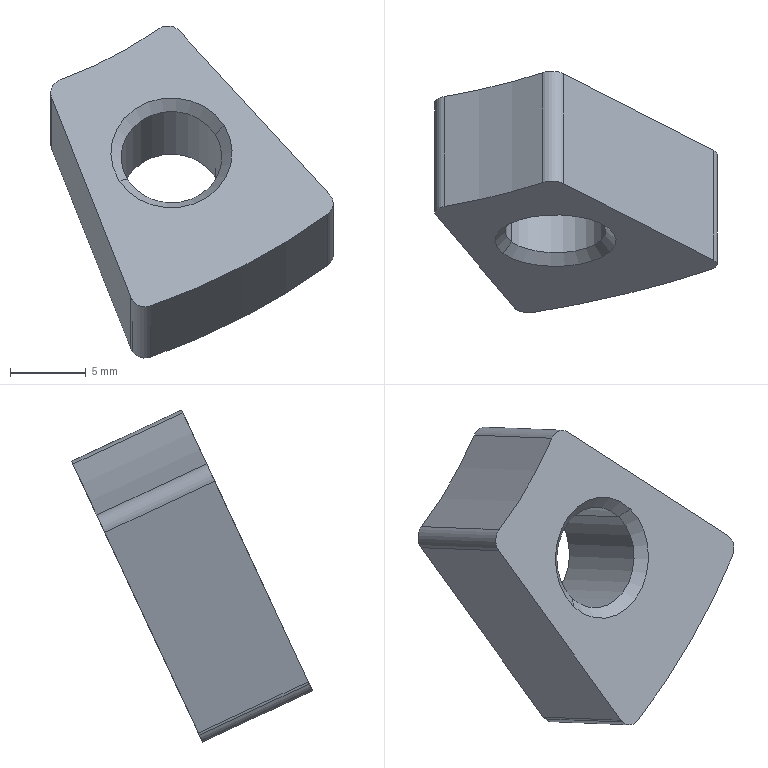Component | SolidWorks | 1369126_DSM_40_270_CC_HD_A_B_0-1_342623_DSM_40_NS-1 | 1 solid | 17 faces | box 18.64 x 15.89 x 21.91 mm | volume 1452 mm3 | cylinder 9 | cone 4 | plane 4 | commonest cylinder face diameters 2 x5 6.647 x2 89 x1 54 x1
build123d program:
from build123d import *

# Parameters (mm, degrees)
BOSS_EXTRUDE1_DEPTH = 8


with BuildPart() as part:
    # Sketch1 → Boss-Extrude1 (new body)
    with BuildSketch(Plane.XY):
        with BuildLine():
            Line((7.552, -7.828), (4.859, 7.443))
            ThreePointArc((4.859, 7.443), (4.462, 8.078), (3.736, 8.26))
            ThreePointArc((3.736, 8.26), (0, 8), (-3.736, 8.26))
            ThreePointArc((-3.736, 8.26), (-4.462, 8.078), (-4.859, 7.443))
            Line((-4.859, 7.443), (-7.552, -7.828))
            ThreePointArc((-7.552, -7.828), (-7.379, -8.584), (-6.718, -8.99))
            ThreePointArc((-6.718, -8.99), (0, -9.5), (6.718, -8.99))
            ThreePointArc((6.718, -8.99), (7.379, -8.584), (7.552, -7.828))
        make_face()
    extrude(amount=BOSS_EXTRUDE1_DEPTH)

    # Sketch2 → Cut-Revolve1 (revolve, cut)
    with BuildSketch(Plane(origin=(0, 0, 0), x_dir=(0, 0, -1), z_dir=(1, 0, 0)), mode=Mode.PRIVATE) as cut_revolve1_sk:
        Polygon((-8, 0), (-8, 4), (-7.324, 3.324), (-0.6765, 3.324), (0, 4), (0, 0), align=None)
    revolve(cut_revolve1_sk.sketch.rotate(Axis((0, 0, 0), (0, 0, 1)), 270), axis=Axis((0, 0, 0), (0, 0, 1)), mode=Mode.SUBTRACT)


solid = part.part

# Placed as in the assembly
solid = solid.moved(Location((-214.207, 2084.435, 247.117), (65, 0, 29.752)))
STEP:
#1=CARTESIAN_POINT('',(-8.547,82.013,9.681));
#2=VERTEX_POINT('',#1);
#3=CARTESIAN_POINT('',(-8.32,82.068,9.799));
#4=VERTEX_POINT('',#3);
#5=CARTESIAN_POINT('',(-8.433,82.04,9.74));
#6=DIRECTION('',(0.,-0.9063,0.4226));
#7=DIRECTION('',(0.8682,0.2097,0.4497));
#8=AXIS2_PLACEMENT_3D('',#5,#6,#7);
#9=CIRCLE('',#8,0.1308);
#10=EDGE_CURVE('',#2,#4,#9,.T.);
#11=ORIENTED_EDGE('',*,*,#10,.T.);
#12=CARTESIAN_POINT('',(-8.297,82.097,9.8));
#13=VERTEX_POINT('',#12);
#14=CARTESIAN_POINT('',(-8.297,82.097,9.8));
#15=DIRECTION('',(0.6139,0.7891,0.01917));
#16=VECTOR('',#15,39.37);
#17=LINE('',#14,#16);
#18=EDGE_CURVE('',#4,#13,#17,.T.);
#19=ORIENTED_EDGE('',*,*,#18,.T.);
#20=CARTESIAN_POINT('',(-8.57,82.031,9.658));
#21=VERTEX_POINT('',#20);
#22=CARTESIAN_POINT('',(-8.433,82.064,9.729));
#23=DIRECTION('',(0.,-0.9063,0.4226));
#24=DIRECTION('',(0.8682,0.2097,0.4497));
#25=AXIS2_PLACEMENT_3D('',#22,#23,#24);
#26=CIRCLE('',#25,0.1575);
#27=EDGE_CURVE('',#21,#13,#26,.T.);
#28=ORIENTED_EDGE('',*,*,#27,.F.);
#29=CARTESIAN_POINT('',(-8.57,82.031,9.658));
#30=DIRECTION('',(-0.6139,0.4926,-0.6168));
#31=VECTOR('',#30,39.37);
#32=LINE('',#29,#31);
#33=EDGE_CURVE('',#2,#21,#32,.T.);
#34=ORIENTED_EDGE('',*,*,#33,.F.);
#35=EDGE_LOOP('',(#11,#19,#28,#34));
#36=FACE_OUTER_BOUND('',#35,.T.);
#37=CARTESIAN_POINT('',(-8.433,82.064,9.729));
#38=DIRECTION('',(-0.,0.9063,-0.4226));
#39=DIRECTION('',(-0.8682,-0.2097,-0.4497));
#40=AXIS2_PLACEMENT_3D('',#37,#38,#39);
#41=CONICAL_SURFACE('',#40,0.1575,0.7854);
#42=ADVANCED_FACE('',(#36),#41,.F.);
#43=ORIENTED_EDGE('',*,*,#10,.F.);
#44=CARTESIAN_POINT('',(-8.547,81.776,9.792));
#45=VERTEX_POINT('',#44);
#46=CARTESIAN_POINT('',(-8.547,82.037,9.67));
#47=DIRECTION('',(0.,-0.9063,0.4226));
#48=VECTOR('',#47,39.37);
#49=LINE('',#46,#48);
#50=EDGE_CURVE('',#2,#45,#49,.T.);
#51=ORIENTED_EDGE('',*,*,#50,.T.);
#52=CARTESIAN_POINT('',(-8.32,81.83,9.91));
#53=VERTEX_POINT('',#52);
#54=CARTESIAN_POINT('',(-8.433,81.803,9.851));
#55=DIRECTION('',(0.,-0.9063,0.4226));
#56=DIRECTION('',(0.8682,0.2097,0.4497));
#57=AXIS2_PLACEMENT_3D('',#54,#55,#56);
#58=CIRCLE('',#57,0.1308);
#59=EDGE_CURVE('',#45,#53,#58,.T.);
#60=ORIENTED_EDGE('',*,*,#59,.T.);
#61=CARTESIAN_POINT('',(-8.32,82.092,9.788));
#62=DIRECTION('',(0.,-0.9063,0.4226));
#63=VECTOR('',#62,39.37);
#64=LINE('',#61,#63);
#65=EDGE_CURVE('',#4,#53,#64,.T.);
#66=ORIENTED_EDGE('',*,*,#65,.F.);
#67=EDGE_LOOP('',(#43,#51,#60,#66));
#68=FACE_OUTER_BOUND('',#67,.T.);
#69=CARTESIAN_POINT('',(-8.433,82.064,9.729));
#70=DIRECTION('',(0.,-0.9063,0.4226));
#71=DIRECTION('',(0.8682,0.2097,0.4497));
#72=AXIS2_PLACEMENT_3D('',#69,#70,#71);
#73=CYLINDRICAL_SURFACE('',#72,0.1308);
#74=ADVANCED_FACE('',(#68),#73,.F.);
#75=ORIENTED_EDGE('',*,*,#59,.F.);
#76=CARTESIAN_POINT('',(-8.57,81.746,9.791));
#77=VERTEX_POINT('',#76);
#78=CARTESIAN_POINT('',(-8.547,81.776,9.792));
#79=DIRECTION('',(-0.6139,-0.7891,-0.01917));
#80=VECTOR('',#79,39.37);
#81=LINE('',#78,#80);
#82=EDGE_CURVE('',#45,#77,#81,.T.);
#83=ORIENTED_EDGE('',*,*,#82,.T.);
#84=CARTESIAN_POINT('',(-8.297,81.812,9.933));
#85=VERTEX_POINT('',#84);
#86=CARTESIAN_POINT('',(-8.433,81.779,9.862));
#87=DIRECTION('',(0.,-0.9063,0.4226));
#88=DIRECTION('',(0.8682,0.2097,0.4497));
#89=AXIS2_PLACEMENT_3D('',#86,#87,#88);
#90=CIRCLE('',#89,0.1575);
#91=EDGE_CURVE('',#77,#85,#90,.T.);
#92=ORIENTED_EDGE('',*,*,#91,.T.);
#93=CARTESIAN_POINT('',(-8.32,81.83,9.91));
#94=DIRECTION('',(0.6139,-0.4926,0.6168));
#95=VECTOR('',#94,39.37);
#96=LINE('',#93,#95);
#97=EDGE_CURVE('',#53,#85,#96,.T.);
#98=ORIENTED_EDGE('',*,*,#97,.F.);
#99=EDGE_LOOP('',(#75,#83,#92,#98));
#100=FACE_OUTER_BOUND('',#99,.T.);
#101=CARTESIAN_POINT('',(-8.433,81.803,9.851));
#102=DIRECTION('',(0.,-0.9063,0.4226));
#103=DIRECTION('',(0.8682,0.2097,0.4497));
#104=AXIS2_PLACEMENT_3D('',#101,#102,#103);
#105=CONICAL_SURFACE('',#104,0.1308,0.7854);
#106=ADVANCED_FACE('',(#100),#105,.F.);
#107=CARTESIAN_POINT('',(-8.536,81.601,9.48));
#108=VERTEX_POINT('',#107);
#109=CARTESIAN_POINT('',(-8.487,81.594,9.465));
#110=VERTEX_POINT('',#109);
#111=CARTESIAN_POINT('',(-8.501,81.609,9.498));
#112=DIRECTION('',(0.,-0.9063,0.4226));
#113=DIRECTION('',(0.8682,0.2097,0.4497));
#114=AXIS2_PLACEMENT_3D('',#111,#112,#113);
#115=CIRCLE('',#114,0.03937);
#116=EDGE_CURVE('',#108,#110,#115,.T.);
#117=ORIENTED_EDGE('',*,*,#116,.F.);
#118=CARTESIAN_POINT('',(-8.536,81.886,9.347));
#119=VERTEX_POINT('',#118);
#120=CARTESIAN_POINT('',(-8.536,81.601,9.48));
#121=DIRECTION('',(-0.,0.9063,-0.4226));
#122=VECTOR('',#121,39.37);
#123=LINE('',#120,#122);
#124=EDGE_CURVE('',#108,#119,#123,.T.);
#125=ORIENTED_EDGE('',*,*,#124,.T.);
#126=CARTESIAN_POINT('',(-8.487,81.879,9.332));
#127=VERTEX_POINT('',#126);
#128=CARTESIAN_POINT('',(-8.501,81.895,9.365));
#129=DIRECTION('',(0.,-0.9063,0.4226));
#130=DIRECTION('',(0.8682,0.2097,0.4497));
#131=AXIS2_PLACEMENT_3D('',#128,#129,#130);
#132=CIRCLE('',#131,0.03937);
#133=EDGE_CURVE('',#119,#127,#132,.T.);
#134=ORIENTED_EDGE('',*,*,#133,.T.);
#135=CARTESIAN_POINT('',(-8.487,81.594,9.465));
#136=DIRECTION('',(-0.,0.9063,-0.4226));
#137=VECTOR('',#136,39.37);
#138=LINE('',#135,#137);
#139=EDGE_CURVE('',#110,#127,#138,.T.);
#140=ORIENTED_EDGE('',*,*,#139,.F.);
#141=EDGE_LOOP('',(#117,#125,#134,#140));
#142=FACE_OUTER_BOUND('',#141,.T.);
#143=CARTESIAN_POINT('',(-8.501,81.609,9.498));
#144=DIRECTION('',(-0.,0.9063,-0.4226));
#145=DIRECTION('',(-0.8682,-0.2097,-0.4497));
#146=AXIS2_PLACEMENT_3D('',#143,#144,#145);
#147=CYLINDRICAL_SURFACE('',#146,0.03937);
#148=ADVANCED_FACE('',(#142),#147,.T.);
#149=ORIENTED_EDGE('',*,*,#124,.F.);
#150=CARTESIAN_POINT('',(-8.539,81.603,9.486));
#151=VERTEX_POINT('',#150);
#152=CARTESIAN_POINT('',(-8.501,81.609,9.498));
#153=DIRECTION('',(0.,-0.9063,0.4226));
#154=DIRECTION('',(0.8682,0.2097,0.4497));
#155=AXIS2_PLACEMENT_3D('',#152,#153,#154);
#156=CIRCLE('',#155,0.03937);
#157=EDGE_CURVE('',#151,#108,#156,.T.);
#158=ORIENTED_EDGE('',*,*,#157,.F.);
#159=CARTESIAN_POINT('',(-8.539,81.889,9.353));
#160=VERTEX_POINT('',#159);
#161=CARTESIAN_POINT('',(-8.539,81.603,9.486));
#162=DIRECTION('',(-0.,0.9063,-0.4226));
#163=VECTOR('',#162,39.37);
#164=LINE('',#161,#163);
#165=EDGE_CURVE('',#151,#160,#164,.T.);
#166=ORIENTED_EDGE('',*,*,#165,.T.);
#167=CARTESIAN_POINT('',(-8.501,81.895,9.365));
#168=DIRECTION('',(0.,-0.9063,0.4226));
#169=DIRECTION('',(0.8682,0.2097,0.4497));
#170=AXIS2_PLACEMENT_3D('',#167,#168,#169);
#171=CIRCLE('',#170,0.03937);
#172=EDGE_CURVE('',#160,#119,#171,.T.);
#173=ORIENTED_EDGE('',*,*,#172,.T.);
#174=EDGE_LOOP('',(#149,#158,#166,#173));
#175=FACE_OUTER_BOUND('',#174,.T.);
#176=CARTESIAN_POINT('',(-8.501,81.609,9.498));
#177=DIRECTION('',(-0.,0.9063,-0.4226));
#178=DIRECTION('',(-0.8682,-0.2097,-0.4497));
#179=AXIS2_PLACEMENT_3D('',#176,#177,#178);
#180=CYLINDRICAL_SURFACE('',#179,0.03937);
#181=ADVANCED_FACE('',(#175),#180,.T.);
#182=CARTESIAN_POINT('',(-8.028,81.99,9.569));
#183=VERTEX_POINT('',#182);
#184=CARTESIAN_POINT('',(-9.117,82.57,10.813));
#185=DIRECTION('',(0.,-0.9063,0.4226));
#186=DIRECTION('',(0.8682,0.2097,0.4497));
#187=AXIS2_PLACEMENT_3D('',#184,#185,#186);
#188=CIRCLE('',#187,1.752);
#189=EDGE_CURVE('',#127,#183,#188,.T.);
#190=ORIENTED_EDGE('',*,*,#189,.T.);
#191=CARTESIAN_POINT('',(-8.028,81.705,9.703));
#192=VERTEX_POINT('',#191);
#193=CARTESIAN_POINT('',(-8.028,81.705,9.703));
#194=DIRECTION('',(-0.,0.9063,-0.4226));
#195=VECTOR('',#194,39.37);
#196=LINE('',#193,#195);
#197=EDGE_CURVE('',#192,#183,#196,.T.);
#198=ORIENTED_EDGE('',*,*,#197,.F.);
#199=CARTESIAN_POINT('',(-9.117,82.285,10.946));
#200=DIRECTION('',(0.,-0.9063,0.4226));
#201=DIRECTION('',(0.8682,0.2097,0.4497));
#202=AXIS2_PLACEMENT_3D('',#199,#200,#201);
#203=CIRCLE('',#202,1.752);
#204=EDGE_CURVE('',#110,#192,#203,.T.);
#205=ORIENTED_EDGE('',*,*,#204,.F.);
#206=ORIENTED_EDGE('',*,*,#139,.T.);
#207=EDGE_LOOP('',(#190,#198,#205,#206));
#208=FACE_OUTER_BOUND('',#207,.T.);
#209=CARTESIAN_POINT('',(-9.117,82.285,10.946));
#210=DIRECTION('',(-0.,0.9063,-0.4226));
#211=DIRECTION('',(-0.8682,-0.2097,-0.4497));
#212=AXIS2_PLACEMENT_3D('',#209,#210,#211);
#213=CYLINDRICAL_SURFACE('',#212,1.752);
#214=ADVANCED_FACE('',(#208),#213,.T.);
#215=CARTESIAN_POINT('',(-8.022,82.014,9.62));
#216=VERTEX_POINT('',#215);
#217=CARTESIAN_POINT('',(-8.053,82.003,9.597));
#218=DIRECTION('',(0.,-0.9063,0.4226));
#219=DIRECTION('',(0.8682,0.2097,0.4497));
#220=AXIS2_PLACEMENT_3D('',#217,#218,#219);
#221=CIRCLE('',#220,0.03937);
#222=EDGE_CURVE('',#183,#216,#221,.T.);
#223=ORIENTED_EDGE('',*,*,#222,.T.);
#224=CARTESIAN_POINT('',(-8.022,81.728,9.753));
#225=VERTEX_POINT('',#224);
#226=CARTESIAN_POINT('',(-8.022,81.728,9.753));
#227=DIRECTION('',(-0.,0.9063,-0.4226));
#228=VECTOR('',#227,39.37);
#229=LINE('',#226,#228);
#230=EDGE_CURVE('',#225,#216,#229,.T.);
#231=ORIENTED_EDGE('',*,*,#230,.F.);
#232=CARTESIAN_POINT('',(-8.053,81.718,9.731));
#233=DIRECTION('',(0.,-0.9063,0.4226));
#234=DIRECTION('',(0.8682,0.2097,0.4497));
#235=AXIS2_PLACEMENT_3D('',#232,#233,#234);
#236=CIRCLE('',#235,0.03937);
#237=EDGE_CURVE('',#192,#225,#236,.T.);
#238=ORIENTED_EDGE('',*,*,#237,.F.);
#239=ORIENTED_EDGE('',*,*,#197,.T.);
#240=EDGE_LOOP('',(#223,#231,#238,#239));
#241=FACE_OUTER_BOUND('',#240,.T.);
#242=CARTESIAN_POINT('',(-8.053,81.718,9.731));
#243=DIRECTION('',(-0.,0.9063,-0.4226));
#244=DIRECTION('',(-0.8682,-0.2097,-0.4497));
#245=AXIS2_PLACEMENT_3D('',#242,#243,#244);
#246=CYLINDRICAL_SURFACE('',#245,0.03937);
#247=ADVANCED_FACE('',(#241),#246,.T.);
#248=CARTESIAN_POINT('',(-8.413,82.212,10.046));
#249=VERTEX_POINT('',#248);
#250=CARTESIAN_POINT('',(-8.022,82.014,9.62));
#251=DIRECTION('',(-0.6394,0.3249,0.6968));
#252=VECTOR('',#251,39.37);
#253=LINE('',#250,#252);
#254=EDGE_CURVE('',#216,#249,#253,.T.);
#255=ORIENTED_EDGE('',*,*,#254,.T.);
#256=CARTESIAN_POINT('',(-8.413,81.927,10.179));
#257=VERTEX_POINT('',#256);
#258=CARTESIAN_POINT('',(-8.413,81.927,10.179));
#259=DIRECTION('',(-0.,0.9063,-0.4226));
#260=VECTOR('',#259,39.37);
#261=LINE('',#258,#260);
#262=EDGE_CURVE('',#257,#249,#261,.T.);
#263=ORIENTED_EDGE('',*,*,#262,.F.);
#264=CARTESIAN_POINT('',(-8.022,81.728,9.753));
#265=DIRECTION('',(-0.6394,0.3249,0.6968));
#266=VECTOR('',#265,39.37);
#267=LINE('',#264,#266);
#268=EDGE_CURVE('',#225,#257,#267,.T.);
#269=ORIENTED_EDGE('',*,*,#268,.F.);
#270=ORIENTED_EDGE('',*,*,#230,.T.);
#271=EDGE_LOOP('',(#255,#263,#269,#270));
#272=FACE_OUTER_BOUND('',#271,.T.);
#273=CARTESIAN_POINT('',(-8.022,81.728,9.753));
#274=DIRECTION('',(-0.7688,-0.2702,-0.5795));
#275=DIRECTION('',(0.6394,-0.3249,-0.6968));
#276=AXIS2_PLACEMENT_3D('',#273,#274,#275);
#277=PLANE('',#276);
#278=ADVANCED_FACE('',(#272),#277,.F.);
#279=CARTESIAN_POINT('',(-8.467,82.215,10.051));
#280=VERTEX_POINT('',#279);
#281=CARTESIAN_POINT('',(-8.443,82.201,10.023));
#282=DIRECTION('',(0.,-0.9063,0.4226));
#283=DIRECTION('',(0.8682,0.2097,0.4497));
#284=AXIS2_PLACEMENT_3D('',#281,#282,#283);
#285=CIRCLE('',#284,0.03937);
#286=EDGE_CURVE('',#249,#280,#285,.T.);
#287=ORIENTED_EDGE('',*,*,#286,.T.);
#288=CARTESIAN_POINT('',(-8.467,81.929,10.184));
#289=VERTEX_POINT('',#288);
#290=CARTESIAN_POINT('',(-8.467,81.929,10.184));
#291=DIRECTION('',(-0.,0.9063,-0.4226));
#292=VECTOR('',#291,39.37);
#293=LINE('',#290,#292);
#294=EDGE_CURVE('',#289,#280,#293,.T.);
#295=ORIENTED_EDGE('',*,*,#294,.F.);
#296=CARTESIAN_POINT('',(-8.443,81.916,10.156));
#297=DIRECTION('',(0.,-0.9063,0.4226));
#298=DIRECTION('',(0.8682,0.2097,0.4497));
#299=AXIS2_PLACEMENT_3D('',#296,#297,#298);
#300=CIRCLE('',#299,0.03937);
#301=EDGE_CURVE('',#257,#289,#300,.T.);
#302=ORIENTED_EDGE('',*,*,#301,.F.);
#303=ORIENTED_EDGE('',*,*,#262,.T.);
#304=EDGE_LOOP('',(#287,#295,#302,#303));
#305=FACE_OUTER_BOUND('',#304,.T.);
#306=CARTESIAN_POINT('',(-8.443,81.916,10.156));
#307=DIRECTION('',(-0.,0.9063,-0.4226));
#308=DIRECTION('',(-0.8682,-0.2097,-0.4497));
#309=AXIS2_PLACEMENT_3D('',#306,#307,#308);
#310=CYLINDRICAL_SURFACE('',#309,0.03937);
#311=ADVANCED_FACE('',(#305),#310,.T.);
#312=CARTESIAN_POINT('',(-8.722,82.153,9.919));
#313=VERTEX_POINT('',#312);
#314=CARTESIAN_POINT('',(-9.117,82.57,10.813));
#315=DIRECTION('',(-0.,0.9063,-0.4226));
#316=DIRECTION('',(-0.8682,-0.2097,-0.4497));
#317=AXIS2_PLACEMENT_3D('',#314,#315,#316);
#318=CIRCLE('',#317,1.063);
#319=EDGE_CURVE('',#280,#313,#318,.T.);
#320=ORIENTED_EDGE('',*,*,#319,.T.);
#321=CARTESIAN_POINT('',(-8.722,81.867,10.052));
#322=VERTEX_POINT('',#321);
#323=CARTESIAN_POINT('',(-8.722,81.867,10.052));
#324=DIRECTION('',(-0.,0.9063,-0.4226));
#325=VECTOR('',#324,39.37);
#326=LINE('',#323,#325);
#327=EDGE_CURVE('',#322,#313,#326,.T.);
#328=ORIENTED_EDGE('',*,*,#327,.F.);
#329=CARTESIAN_POINT('',(-9.117,82.285,10.946));
#330=DIRECTION('',(-0.,0.9063,-0.4226));
#331=DIRECTION('',(-0.8682,-0.2097,-0.4497));
#332=AXIS2_PLACEMENT_3D('',#329,#330,#331);
#333=CIRCLE('',#332,1.063);
#334=EDGE_CURVE('',#289,#322,#333,.T.);
#335=ORIENTED_EDGE('',*,*,#334,.F.);
#336=ORIENTED_EDGE('',*,*,#294,.T.);
#337=EDGE_LOOP('',(#320,#328,#335,#336));
#338=FACE_OUTER_BOUND('',#337,.T.);
#339=CARTESIAN_POINT('',(-9.117,82.285,10.946));
#340=DIRECTION('',(-0.,0.9063,-0.4226));
#341=DIRECTION('',(-0.8682,-0.2097,-0.4497));
#342=AXIS2_PLACEMENT_3D('',#339,#340,#341);
#343=CYLINDRICAL_SURFACE('',#342,1.063);
#344=ADVANCED_FACE('',(#338),#343,.F.);
#345=CARTESIAN_POINT('',(-8.745,82.132,9.874));
#346=VERTEX_POINT('',#345);
#347=CARTESIAN_POINT('',(-8.708,82.137,9.886));
#348=DIRECTION('',(0.,-0.9063,0.4226));
#349=DIRECTION('',(0.8682,0.2097,0.4497));
#350=AXIS2_PLACEMENT_3D('',#347,#348,#349);
#351=CIRCLE('',#350,0.03937);
#352=EDGE_CURVE('',#313,#346,#351,.T.);
#353=ORIENTED_EDGE('',*,*,#352,.T.);
#354=CARTESIAN_POINT('',(-8.745,81.846,10.007));
#355=VERTEX_POINT('',#354);
#356=CARTESIAN_POINT('',(-8.745,81.846,10.007));
#357=DIRECTION('',(-0.,0.9063,-0.4226));
#358=VECTOR('',#357,39.37);
#359=LINE('',#356,#358);
#360=EDGE_CURVE('',#355,#346,#359,.T.);
#361=ORIENTED_EDGE('',*,*,#360,.F.);
#362=CARTESIAN_POINT('',(-8.708,81.852,10.019));
#363=DIRECTION('',(0.,-0.9063,0.4226));
#364=DIRECTION('',(0.8682,0.2097,0.4497));
#365=AXIS2_PLACEMENT_3D('',#362,#363,#364);
#366=CIRCLE('',#365,0.03937);
#367=EDGE_CURVE('',#322,#355,#366,.T.);
#368=ORIENTED_EDGE('',*,*,#367,.F.);
#369=ORIENTED_EDGE('',*,*,#327,.T.);
#370=EDGE_LOOP('',(#353,#361,#368,#369));
#371=FACE_OUTER_BOUND('',#370,.T.);
#372=CARTESIAN_POINT('',(-8.708,81.852,10.019));
#373=DIRECTION('',(-0.,0.9063,-0.4226));
#374=DIRECTION('',(-0.8682,-0.2097,-0.4497));
#375=AXIS2_PLACEMENT_3D('',#372,#373,#374);
#376=CYLINDRICAL_SURFACE('',#375,0.03937);
#377=ADVANCED_FACE('',(#371),#376,.T.);
#378=CARTESIAN_POINT('',(-8.745,82.132,9.874));
#379=DIRECTION('',(0.3379,-0.3978,-0.853));
#380=VECTOR('',#379,39.37);
#381=LINE('',#378,#380);
#382=EDGE_CURVE('',#346,#160,#381,.T.);
#383=ORIENTED_EDGE('',*,*,#382,.T.);
#384=ORIENTED_EDGE('',*,*,#165,.F.);
#385=CARTESIAN_POINT('',(-8.745,81.846,10.007));
#386=DIRECTION('',(0.3379,-0.3978,-0.853));
#387=VECTOR('',#386,39.37);
#388=LINE('',#385,#387);
#389=EDGE_CURVE('',#355,#151,#388,.T.);
#390=ORIENTED_EDGE('',*,*,#389,.F.);
#391=ORIENTED_EDGE('',*,*,#360,.T.);
#392=EDGE_LOOP('',(#383,#384,#390,#391));
#393=FACE_OUTER_BOUND('',#392,.T.);
#394=CARTESIAN_POINT('',(-8.745,81.846,10.007));
#395=DIRECTION('',(0.9412,0.1428,0.3063));
#396=DIRECTION('',(-0.3379,0.3978,0.853));
#397=AXIS2_PLACEMENT_3D('',#394,#395,#396);
#398=PLANE('',#397);
#399=ADVANCED_FACE('',(#393),#398,.F.);
#400=CARTESIAN_POINT('',(-8.433,81.779,9.862));
#401=DIRECTION('',(0.,-0.9063,0.4226));
#402=DIRECTION('',(0.8682,0.2097,0.4497));
#403=AXIS2_PLACEMENT_3D('',#400,#401,#402);
#404=CIRCLE('',#403,0.1575);
#405=EDGE_CURVE('',#85,#77,#404,.T.);
#406=ORIENTED_EDGE('',*,*,#405,.F.);
#407=ORIENTED_EDGE('',*,*,#91,.F.);
#408=EDGE_LOOP('',(#406,#407));
#409=FACE_BOUND('',#408,.T.);
#410=ORIENTED_EDGE('',*,*,#157,.T.);
#411=ORIENTED_EDGE('',*,*,#116,.T.);
#412=ORIENTED_EDGE('',*,*,#204,.T.);
#413=ORIENTED_EDGE('',*,*,#237,.T.);
#414=ORIENTED_EDGE('',*,*,#268,.T.);
#415=ORIENTED_EDGE('',*,*,#301,.T.);
#416=ORIENTED_EDGE('',*,*,#334,.T.);
#417=ORIENTED_EDGE('',*,*,#367,.T.);
#418=ORIENTED_EDGE('',*,*,#389,.T.);
#419=EDGE_LOOP('',(#410,#411,#412,#413,#414,#415,#416,#417,#418));
#420=FACE_OUTER_BOUND('',#419,.T.);
#421=CARTESIAN_POINT('',(-8.501,81.609,9.498));
#422=DIRECTION('',(0.,-0.9063,0.4226));
#423=DIRECTION('',(0.8682,0.2097,0.4497));
#424=AXIS2_PLACEMENT_3D('',#421,#422,#423);
#425=PLANE('',#424);
#426=ADVANCED_FACE('',(#409,#420),#425,.T.);
#427=ORIENTED_EDGE('',*,*,#27,.T.);
#428=CARTESIAN_POINT('',(-8.433,82.064,9.729));
#429=DIRECTION('',(0.,-0.9063,0.4226));
#430=DIRECTION('',(0.8682,0.2097,0.4497));
#431=AXIS2_PLACEMENT_3D('',#428,#429,#430);
#432=CIRCLE('',#431,0.1575);
#433=EDGE_CURVE('',#13,#21,#432,.T.);
#434=ORIENTED_EDGE('',*,*,#433,.T.);
#435=EDGE_LOOP('',(#427,#434));
#436=FACE_BOUND('',#435,.T.);
#437=ORIENTED_EDGE('',*,*,#172,.F.);
#438=ORIENTED_EDGE('',*,*,#382,.F.);
#439=ORIENTED_EDGE('',*,*,#352,.F.);
#440=ORIENTED_EDGE('',*,*,#319,.F.);
#441=ORIENTED_EDGE('',*,*,#286,.F.);
#442=ORIENTED_EDGE('',*,*,#254,.F.);
#443=ORIENTED_EDGE('',*,*,#222,.F.);
#444=ORIENTED_EDGE('',*,*,#189,.F.);
#445=ORIENTED_EDGE('',*,*,#133,.F.);
#446=EDGE_LOOP('',(#437,#438,#439,#440,#441,#442,#443,#444,#445));
#447=FACE_OUTER_BOUND('',#446,.T.);
#448=CARTESIAN_POINT('',(-8.501,81.895,9.365));
#449=DIRECTION('',(0.,-0.9063,0.4226));
#450=DIRECTION('',(0.8682,0.2097,0.4497));
#451=AXIS2_PLACEMENT_3D('',#448,#449,#450);
#452=PLANE('',#451);
#453=ADVANCED_FACE('',(#436,#447),#452,.F.);
#454=ORIENTED_EDGE('',*,*,#82,.F.);
#455=CARTESIAN_POINT('',(-8.433,81.803,9.851));
#456=DIRECTION('',(0.,-0.9063,0.4226));
#457=DIRECTION('',(0.8682,0.2097,0.4497));
#458=AXIS2_PLACEMENT_3D('',#455,#456,#457);
#459=CIRCLE('',#458,0.1308);
#460=EDGE_CURVE('',#53,#45,#459,.T.);
#461=ORIENTED_EDGE('',*,*,#460,.F.);
#462=ORIENTED_EDGE('',*,*,#97,.T.);
#463=ORIENTED_EDGE('',*,*,#405,.T.);
#464=EDGE_LOOP('',(#454,#461,#462,#463));
#465=FACE_OUTER_BOUND('',#464,.T.);
#466=CARTESIAN_POINT('',(-8.433,81.803,9.851));
#467=DIRECTION('',(0.,-0.9063,0.4226));
#468=DIRECTION('',(0.8682,0.2097,0.4497));
#469=AXIS2_PLACEMENT_3D('',#466,#467,#468);
#470=CONICAL_SURFACE('',#469,0.1308,0.7854);
#471=ADVANCED_FACE('',(#465),#470,.F.);
#472=ORIENTED_EDGE('',*,*,#50,.F.);
#473=CARTESIAN_POINT('',(-8.433,82.04,9.74));
#474=DIRECTION('',(0.,-0.9063,0.4226));
#475=DIRECTION('',(0.8682,0.2097,0.4497));
#476=AXIS2_PLACEMENT_3D('',#473,#474,#475);
#477=CIRCLE('',#476,0.1308);
#478=EDGE_CURVE('',#4,#2,#477,.T.);
#479=ORIENTED_EDGE('',*,*,#478,.F.);
#480=ORIENTED_EDGE('',*,*,#65,.T.);
#481=ORIENTED_EDGE('',*,*,#460,.T.);
#482=EDGE_LOOP('',(#472,#479,#480,#481));
#483=FACE_OUTER_BOUND('',#482,.T.);
#484=CARTESIAN_POINT('',(-8.433,82.064,9.729));
#485=DIRECTION('',(0.,-0.9063,0.4226));
#486=DIRECTION('',(0.8682,0.2097,0.4497));
#487=AXIS2_PLACEMENT_3D('',#484,#485,#486);
#488=CYLINDRICAL_SURFACE('',#487,0.1308);
#489=ADVANCED_FACE('',(#483),#488,.F.);
#490=ORIENTED_EDGE('',*,*,#18,.F.);
#491=ORIENTED_EDGE('',*,*,#478,.T.);
#492=ORIENTED_EDGE('',*,*,#33,.T.);
#493=ORIENTED_EDGE('',*,*,#433,.F.);
#494=EDGE_LOOP('',(#490,#491,#492,#493));
#495=FACE_OUTER_BOUND('',#494,.T.);
#496=CARTESIAN_POINT('',(-8.433,82.064,9.729));
#497=DIRECTION('',(-0.,0.9063,-0.4226));
#498=DIRECTION('',(-0.8682,-0.2097,-0.4497));
#499=AXIS2_PLACEMENT_3D('',#496,#497,#498);
#500=CONICAL_SURFACE('',#499,0.1575,0.7854);
#501=ADVANCED_FACE('',(#495),#500,.F.);
#502=CLOSED_SHELL('',(#42,#74,#106,#148,#181,#214,#247,#278,#311,#344,#377,#399,#426,#453,#471,#489,#501));
#503=MANIFOLD_SOLID_BREP('',#502);
#504=CARTESIAN_POINT('',(0.,0.,0.));
#505=DIRECTION('',(0.,0.,1.));
#506=DIRECTION('',(1.,0.,0.));
#507=AXIS2_PLACEMENT_3D('',#504,#505,#506);
#508=(LENGTH_UNIT()NAMED_UNIT(*)SI_UNIT($,.METRE.));
#509=LENGTH_MEASURE_WITH_UNIT(LENGTH_MEASURE(0.0254),#508);
#510=DIMENSIONAL_EXPONENTS(1.,0.,0.,0.,0.,0.,0.);
#511=(CONVERSION_BASED_UNIT('',#509)LENGTH_UNIT()NAMED_UNIT(#510));
#512=UNCERTAINTY_MEASURE_WITH_UNIT(LENGTH_MEASURE(0.00001),#511,'','');
#513=(NAMED_UNIT(*)PLANE_ANGLE_UNIT()SI_UNIT($,.RADIAN.));
#514=(NAMED_UNIT(*)SI_UNIT($,.STERADIAN.)SOLID_ANGLE_UNIT());
#515=(GEOMETRIC_REPRESENTATION_CONTEXT(3)GLOBAL_UNCERTAINTY_ASSIGNED_CONTEXT((#512))GLOBAL_UNIT_ASSIGNED_CONTEXT((#511,#513,#514))REPRESENTATION_CONTEXT('',''));
#516=ADVANCED_BREP_SHAPE_REPRESENTATION('',(#503,#507),#515);
#517=COLOUR_RGB('',0.7922,0.8196,0.9333);
#518=FILL_AREA_STYLE_COLOUR('',#517);
#519=FILL_AREA_STYLE('',(#518));
#520=SURFACE_STYLE_FILL_AREA(#519);
#521=SURFACE_SIDE_STYLE('',(#520));
#522=SURFACE_STYLE_USAGE(.BOTH.,#521);
#523=PRESENTATION_STYLE_ASSIGNMENT((#522));
#524=STYLED_ITEM('',(#523),#503);
#525=(LENGTH_UNIT()NAMED_UNIT(*)SI_UNIT($,.METRE.));
#526=LENGTH_MEASURE_WITH_UNIT(LENGTH_MEASURE(0.0254),#525);
#527=DIMENSIONAL_EXPONENTS(1.,0.,0.,0.,0.,0.,0.);
#528=(CONVERSION_BASED_UNIT('',#526)LENGTH_UNIT()NAMED_UNIT(#527));
#529=UNCERTAINTY_MEASURE_WITH_UNIT(LENGTH_MEASURE(0.00001),#528,'','');
#530=(NAMED_UNIT(*)PLANE_ANGLE_UNIT()SI_UNIT($,.RADIAN.));
#531=(NAMED_UNIT(*)SI_UNIT($,.STERADIAN.)SOLID_ANGLE_UNIT());
#532=(GEOMETRIC_REPRESENTATION_CONTEXT(3)GLOBAL_UNCERTAINTY_ASSIGNED_CONTEXT((#529))GLOBAL_UNIT_ASSIGNED_CONTEXT((#528,#530,#531))REPRESENTATION_CONTEXT('',''));
#533=MECHANICAL_DESIGN_GEOMETRIC_PRESENTATION_REPRESENTATION('',(#524),#532);
#534=PRESENTATION_LAYER_ASSIGNMENT('','',(#524));